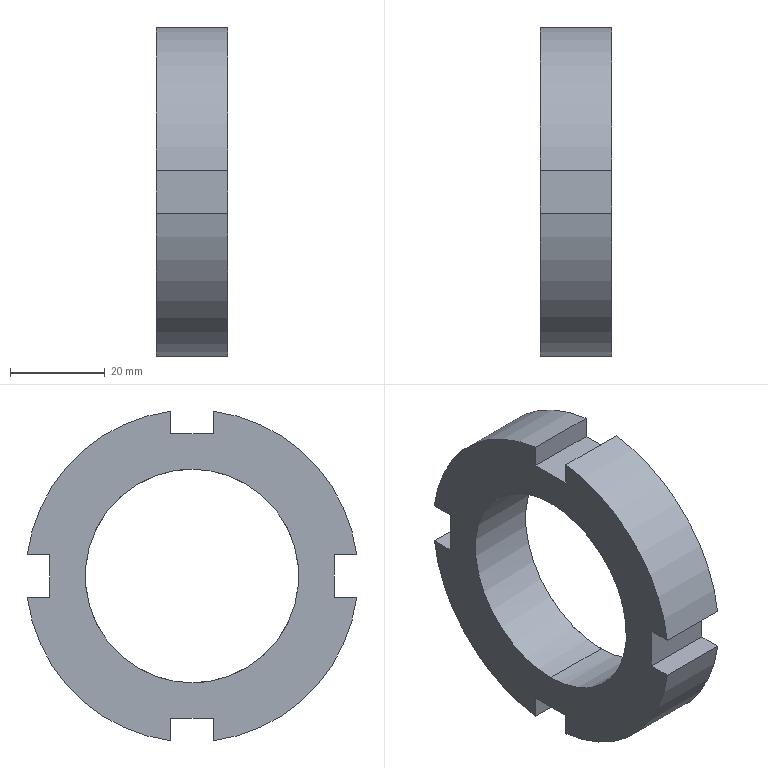Component | SolidWorks | 5Nut-1 | 1 solid | 22 faces | box 15 x 69.42 x 69.42 mm | volume 31223 mm3 | plane 14 | cylinder 6 | cone 2 | commonest cylinder face diameters 70 x4 45 x2
STEP:
#1=COLOUR_RGB('',0.7922,0.8196,0.9333);
#2=FILL_AREA_STYLE_COLOUR('',#1);
#3=FILL_AREA_STYLE('',(#2));
#4=SURFACE_STYLE_FILL_AREA(#3);
#5=SURFACE_SIDE_STYLE('',(#4));
#6=SURFACE_STYLE_USAGE(.BOTH.,#5);
#7=PRESENTATION_STYLE_ASSIGNMENT((#6));
#8=CARTESIAN_POINT('',(-5.674,-3.551,21.043));
#9=VERTEX_POINT('',#8);
#10=CARTESIAN_POINT('',(-5.674,-3.551,19.272));
#11=VERTEX_POINT('',#10);
#12=CARTESIAN_POINT('',(-5.674,-3.551,21.043));
#13=CARTESIAN_POINT('',(-5.674,-3.609,21.043));
#14=CARTESIAN_POINT('',(-5.674,-3.667,21.038));
#15=CARTESIAN_POINT('',(-5.674,-3.781,21.015));
#16=CARTESIAN_POINT('',(-5.674,-3.836,20.998));
#17=CARTESIAN_POINT('',(-5.674,-3.944,20.954));
#18=CARTESIAN_POINT('',(-5.674,-3.995,20.926));
#19=CARTESIAN_POINT('',(-5.674,-4.091,20.862));
#20=CARTESIAN_POINT('',(-5.674,-4.136,20.825));
#21=CARTESIAN_POINT('',(-5.674,-4.218,20.743));
#22=CARTESIAN_POINT('',(-5.674,-4.255,20.698));
#23=CARTESIAN_POINT('',(-5.674,-4.32,20.601));
#24=CARTESIAN_POINT('',(-5.674,-4.347,20.55));
#25=CARTESIAN_POINT('',(-5.674,-4.391,20.443));
#26=CARTESIAN_POINT('',(-5.674,-4.408,20.387));
#27=CARTESIAN_POINT('',(-5.674,-4.431,20.273));
#28=CARTESIAN_POINT('',(-5.674,-4.437,20.216));
#29=CARTESIAN_POINT('',(-5.674,-4.437,20.099));
#30=CARTESIAN_POINT('',(-5.674,-4.431,20.042));
#31=CARTESIAN_POINT('',(-5.674,-4.408,19.928));
#32=CARTESIAN_POINT('',(-5.674,-4.391,19.872));
#33=CARTESIAN_POINT('',(-5.674,-4.347,19.765));
#34=CARTESIAN_POINT('',(-5.674,-4.32,19.714));
#35=CARTESIAN_POINT('',(-5.674,-4.255,19.617));
#36=CARTESIAN_POINT('',(-5.674,-4.218,19.572));
#37=CARTESIAN_POINT('',(-5.674,-4.136,19.49));
#38=CARTESIAN_POINT('',(-5.674,-4.091,19.453));
#39=CARTESIAN_POINT('',(-5.674,-3.995,19.389));
#40=CARTESIAN_POINT('',(-5.674,-3.944,19.361));
#41=CARTESIAN_POINT('',(-5.674,-3.836,19.317));
#42=CARTESIAN_POINT('',(-5.674,-3.781,19.3));
#43=CARTESIAN_POINT('',(-5.674,-3.667,19.277));
#44=CARTESIAN_POINT('',(-5.674,-3.609,19.272));
#45=CARTESIAN_POINT('',(-5.674,-3.551,19.272));
#46=B_SPLINE_CURVE_WITH_KNOTS('',3,(#12,#13,#14,#15,#16,#17,#18,#19,#20,#21,#22,#23,#24,#25,#26,#27,#28,#29,#30,#31,#32,#33,#34,#35,#36,#37,#38,#39,#40,#41,#42,#43,#44,#45),.UNSPECIFIED.,.F.,.F.,(4,2,2,2,2,2,2,2,2,2,2,2,2,2,2,2,4),(0.5,0.5312,0.5625,0.5938,0.625,0.6562,0.6875,0.7188,0.75,0.7812,0.8125,0.8438,0.875,0.9062,0.9375,0.9688,1.),.UNSPECIFIED.);
#47=EDGE_CURVE('',#9,#11,#46,.T.);
#48=ORIENTED_EDGE('',*,*,#47,.F.);
#49=CARTESIAN_POINT('',(-5.084,-3.551,21.043));
#50=VERTEX_POINT('',#49);
#51=CARTESIAN_POINT('',(-5.674,-3.551,21.043));
#52=DIRECTION('',(1.,0.,0.));
#53=VECTOR('',#52,39.37);
#54=LINE('',#51,#53);
#55=EDGE_CURVE('',#9,#50,#54,.T.);
#56=ORIENTED_EDGE('',*,*,#55,.T.);
#57=CARTESIAN_POINT('',(-5.084,-3.551,19.272));
#58=VERTEX_POINT('',#57);
#59=CARTESIAN_POINT('',(-5.084,-3.551,20.157));
#60=DIRECTION('',(-1.,0.,0.));
#61=DIRECTION('',(0.,0.,-1.));
#62=AXIS2_PLACEMENT_3D('',#59,#60,#61);
#63=CIRCLE('',#62,0.8858);
#64=EDGE_CURVE('',#58,#50,#63,.T.);
#65=ORIENTED_EDGE('',*,*,#64,.F.);
#66=CARTESIAN_POINT('',(-5.674,-3.551,19.272));
#67=DIRECTION('',(1.,0.,0.));
#68=VECTOR('',#67,39.37);
#69=LINE('',#66,#68);
#70=EDGE_CURVE('',#11,#58,#69,.T.);
#71=ORIENTED_EDGE('',*,*,#70,.F.);
#72=EDGE_LOOP('',(#48,#56,#65,#71));
#73=FACE_OUTER_BOUND('',#72,.T.);
#74=CARTESIAN_POINT('',(-5.674,-3.551,20.157));
#75=DIRECTION('',(1.,0.,0.));
#76=DIRECTION('',(0.,0.,-1.));
#77=AXIS2_PLACEMENT_3D('',#74,#75,#76);
#78=CYLINDRICAL_SURFACE('',#77,0.8858);
#79=ADVANCED_FACE('',(#73),#78,.F.);
#80=ORIENTED_EDGE('',*,*,#64,.T.);
#81=CARTESIAN_POINT('',(-5.083,-3.551,21.044));
#82=VERTEX_POINT('',#81);
#83=CARTESIAN_POINT('',(-5.083,-3.551,21.044));
#84=DIRECTION('',(0.7071,0.,0.7071));
#85=VECTOR('',#84,39.37);
#86=LINE('',#83,#85);
#87=EDGE_CURVE('',#50,#82,#86,.T.);
#88=ORIENTED_EDGE('',*,*,#87,.T.);
#89=CARTESIAN_POINT('',(-5.083,-3.551,19.271));
#90=VERTEX_POINT('',#89);
#91=CARTESIAN_POINT('',(-5.083,-3.551,20.157));
#92=DIRECTION('',(1.,0.,0.));
#93=DIRECTION('',(0.,0.,-1.));
#94=AXIS2_PLACEMENT_3D('',#91,#92,#93);
#95=CIRCLE('',#94,0.8868);
#96=EDGE_CURVE('',#82,#90,#95,.T.);
#97=ORIENTED_EDGE('',*,*,#96,.T.);
#98=CARTESIAN_POINT('',(-5.083,-3.551,19.271));
#99=DIRECTION('',(0.7071,0.,-0.7071));
#100=VECTOR('',#99,39.37);
#101=LINE('',#98,#100);
#102=EDGE_CURVE('',#58,#90,#101,.T.);
#103=ORIENTED_EDGE('',*,*,#102,.F.);
#104=EDGE_LOOP('',(#80,#88,#97,#103));
#105=FACE_OUTER_BOUND('',#104,.T.);
#106=CARTESIAN_POINT('',(-5.083,-3.551,20.157));
#107=DIRECTION('',(1.,0.,0.));
#108=DIRECTION('',(0.,0.,-1.));
#109=AXIS2_PLACEMENT_3D('',#106,#107,#108);
#110=CONICAL_SURFACE('',#109,0.8868,0.7854);
#111=ADVANCED_FACE('',(#105),#110,.F.);
#112=CARTESIAN_POINT('',(-5.674,-2.184,19.98));
#113=VERTEX_POINT('',#112);
#114=CARTESIAN_POINT('',(-5.083,-2.184,19.98));
#115=VERTEX_POINT('',#114);
#116=CARTESIAN_POINT('',(-5.674,-2.184,19.98));
#117=DIRECTION('',(1.,0.,0.));
#118=VECTOR('',#117,39.37);
#119=LINE('',#116,#118);
#120=EDGE_CURVE('',#113,#115,#119,.T.);
#121=ORIENTED_EDGE('',*,*,#120,.T.);
#122=CARTESIAN_POINT('',(-5.083,-3.374,18.791));
#123=VERTEX_POINT('',#122);
#124=CARTESIAN_POINT('',(-5.083,-3.551,20.157));
#125=DIRECTION('',(1.,0.,0.));
#126=DIRECTION('',(0.,0.,-1.));
#127=AXIS2_PLACEMENT_3D('',#124,#125,#126);
#128=CIRCLE('',#127,1.378);
#129=EDGE_CURVE('',#123,#115,#128,.T.);
#130=ORIENTED_EDGE('',*,*,#129,.F.);
#131=CARTESIAN_POINT('',(-5.674,-3.374,18.791));
#132=VERTEX_POINT('',#131);
#133=CARTESIAN_POINT('',(-5.674,-3.374,18.791));
#134=DIRECTION('',(1.,0.,0.));
#135=VECTOR('',#134,39.37);
#136=LINE('',#133,#135);
#137=EDGE_CURVE('',#132,#123,#136,.T.);
#138=ORIENTED_EDGE('',*,*,#137,.F.);
#139=CARTESIAN_POINT('',(-5.674,-3.551,20.157));
#140=DIRECTION('',(1.,0.,0.));
#141=DIRECTION('',(0.,0.,-1.));
#142=AXIS2_PLACEMENT_3D('',#139,#140,#141);
#143=CIRCLE('',#142,1.378);
#144=EDGE_CURVE('',#132,#113,#143,.T.);
#145=ORIENTED_EDGE('',*,*,#144,.T.);
#146=EDGE_LOOP('',(#121,#130,#138,#145));
#147=FACE_OUTER_BOUND('',#146,.T.);
#148=CARTESIAN_POINT('',(-5.083,-3.551,20.157));
#149=DIRECTION('',(-1.,0.,0.));
#150=DIRECTION('',(0.,0.,1.));
#151=AXIS2_PLACEMENT_3D('',#148,#149,#150);
#152=CYLINDRICAL_SURFACE('',#151,1.378);
#153=ADVANCED_FACE('',(#147),#152,.T.);
#154=CARTESIAN_POINT('',(-5.083,-2.184,20.335));
#155=VERTEX_POINT('',#154);
#156=CARTESIAN_POINT('',(-5.083,-3.374,21.524));
#157=VERTEX_POINT('',#156);
#158=CARTESIAN_POINT('',(-5.083,-3.551,20.157));
#159=DIRECTION('',(1.,0.,0.));
#160=DIRECTION('',(0.,0.,-1.));
#161=AXIS2_PLACEMENT_3D('',#158,#159,#160);
#162=CIRCLE('',#161,1.378);
#163=EDGE_CURVE('',#155,#157,#162,.T.);
#164=ORIENTED_EDGE('',*,*,#163,.F.);
#165=CARTESIAN_POINT('',(-5.674,-2.184,20.335));
#166=VERTEX_POINT('',#165);
#167=CARTESIAN_POINT('',(-5.674,-2.184,20.335));
#168=DIRECTION('',(1.,0.,0.));
#169=VECTOR('',#168,39.37);
#170=LINE('',#167,#169);
#171=EDGE_CURVE('',#166,#155,#170,.T.);
#172=ORIENTED_EDGE('',*,*,#171,.F.);
#173=CARTESIAN_POINT('',(-5.674,-3.374,21.524));
#174=VERTEX_POINT('',#173);
#175=CARTESIAN_POINT('',(-5.674,-3.551,20.157));
#176=DIRECTION('',(1.,0.,0.));
#177=DIRECTION('',(0.,0.,-1.));
#178=AXIS2_PLACEMENT_3D('',#175,#176,#177);
#179=CIRCLE('',#178,1.378);
#180=EDGE_CURVE('',#166,#174,#179,.T.);
#181=ORIENTED_EDGE('',*,*,#180,.T.);
#182=CARTESIAN_POINT('',(-5.674,-3.374,21.524));
#183=DIRECTION('',(1.,0.,0.));
#184=VECTOR('',#183,39.37);
#185=LINE('',#182,#184);
#186=EDGE_CURVE('',#174,#157,#185,.T.);
#187=ORIENTED_EDGE('',*,*,#186,.T.);
#188=EDGE_LOOP('',(#164,#172,#181,#187));
#189=FACE_OUTER_BOUND('',#188,.T.);
#190=CARTESIAN_POINT('',(-5.083,-3.551,20.157));
#191=DIRECTION('',(-1.,0.,0.));
#192=DIRECTION('',(0.,0.,1.));
#193=AXIS2_PLACEMENT_3D('',#190,#191,#192);
#194=CYLINDRICAL_SURFACE('',#193,1.378);
#195=ADVANCED_FACE('',(#189),#194,.T.);
#196=CARTESIAN_POINT('',(-5.083,-3.728,21.524));
#197=VERTEX_POINT('',#196);
#198=CARTESIAN_POINT('',(-5.083,-4.917,20.335));
#199=VERTEX_POINT('',#198);
#200=CARTESIAN_POINT('',(-5.083,-3.551,20.157));
#201=DIRECTION('',(1.,0.,0.));
#202=DIRECTION('',(0.,0.,-1.));
#203=AXIS2_PLACEMENT_3D('',#200,#201,#202);
#204=CIRCLE('',#203,1.378);
#205=EDGE_CURVE('',#197,#199,#204,.T.);
#206=ORIENTED_EDGE('',*,*,#205,.F.);
#207=CARTESIAN_POINT('',(-5.674,-3.728,21.524));
#208=VERTEX_POINT('',#207);
#209=CARTESIAN_POINT('',(-5.674,-3.728,21.524));
#210=DIRECTION('',(1.,0.,0.));
#211=VECTOR('',#210,39.37);
#212=LINE('',#209,#211);
#213=EDGE_CURVE('',#208,#197,#212,.T.);
#214=ORIENTED_EDGE('',*,*,#213,.F.);
#215=CARTESIAN_POINT('',(-5.674,-4.917,20.335));
#216=VERTEX_POINT('',#215);
#217=CARTESIAN_POINT('',(-5.674,-3.551,20.157));
#218=DIRECTION('',(1.,0.,0.));
#219=DIRECTION('',(0.,0.,-1.));
#220=AXIS2_PLACEMENT_3D('',#217,#218,#219);
#221=CIRCLE('',#220,1.378);
#222=EDGE_CURVE('',#208,#216,#221,.T.);
#223=ORIENTED_EDGE('',*,*,#222,.T.);
#224=CARTESIAN_POINT('',(-5.674,-4.917,20.335));
#225=DIRECTION('',(1.,0.,0.));
#226=VECTOR('',#225,39.37);
#227=LINE('',#224,#226);
#228=EDGE_CURVE('',#216,#199,#227,.T.);
#229=ORIENTED_EDGE('',*,*,#228,.T.);
#230=EDGE_LOOP('',(#206,#214,#223,#229));
#231=FACE_OUTER_BOUND('',#230,.T.);
#232=CARTESIAN_POINT('',(-5.083,-3.551,20.157));
#233=DIRECTION('',(-1.,0.,0.));
#234=DIRECTION('',(0.,0.,1.));
#235=AXIS2_PLACEMENT_3D('',#232,#233,#234);
#236=CYLINDRICAL_SURFACE('',#235,1.378);
#237=ADVANCED_FACE('',(#231),#236,.T.);
#238=CARTESIAN_POINT('',(-5.083,-4.917,19.98));
#239=VERTEX_POINT('',#238);
#240=CARTESIAN_POINT('',(-5.083,-3.728,18.791));
#241=VERTEX_POINT('',#240);
#242=CARTESIAN_POINT('',(-5.083,-3.551,20.157));
#243=DIRECTION('',(1.,0.,0.));
#244=DIRECTION('',(0.,0.,-1.));
#245=AXIS2_PLACEMENT_3D('',#242,#243,#244);
#246=CIRCLE('',#245,1.378);
#247=EDGE_CURVE('',#239,#241,#246,.T.);
#248=ORIENTED_EDGE('',*,*,#247,.F.);
#249=CARTESIAN_POINT('',(-5.674,-4.917,19.98));
#250=VERTEX_POINT('',#249);
#251=CARTESIAN_POINT('',(-5.674,-4.917,19.98));
#252=DIRECTION('',(1.,0.,0.));
#253=VECTOR('',#252,39.37);
#254=LINE('',#251,#253);
#255=EDGE_CURVE('',#250,#239,#254,.T.);
#256=ORIENTED_EDGE('',*,*,#255,.F.);
#257=CARTESIAN_POINT('',(-5.674,-3.728,18.791));
#258=VERTEX_POINT('',#257);
#259=CARTESIAN_POINT('',(-5.674,-3.551,20.157));
#260=DIRECTION('',(1.,0.,0.));
#261=DIRECTION('',(0.,0.,-1.));
#262=AXIS2_PLACEMENT_3D('',#259,#260,#261);
#263=CIRCLE('',#262,1.378);
#264=EDGE_CURVE('',#250,#258,#263,.T.);
#265=ORIENTED_EDGE('',*,*,#264,.T.);
#266=CARTESIAN_POINT('',(-5.674,-3.728,18.791));
#267=DIRECTION('',(1.,0.,0.));
#268=VECTOR('',#267,39.37);
#269=LINE('',#266,#268);
#270=EDGE_CURVE('',#258,#241,#269,.T.);
#271=ORIENTED_EDGE('',*,*,#270,.T.);
#272=EDGE_LOOP('',(#248,#256,#265,#271));
#273=FACE_OUTER_BOUND('',#272,.T.);
#274=CARTESIAN_POINT('',(-5.083,-3.551,20.157));
#275=DIRECTION('',(-1.,0.,0.));
#276=DIRECTION('',(0.,0.,1.));
#277=AXIS2_PLACEMENT_3D('',#274,#275,#276);
#278=CYLINDRICAL_SURFACE('',#277,1.378);
#279=ADVANCED_FACE('',(#273),#278,.T.);
#280=CARTESIAN_POINT('',(-5.083,-3.551,20.157));
#281=DIRECTION('',(1.,0.,0.));
#282=DIRECTION('',(0.,0.,-1.));
#283=AXIS2_PLACEMENT_3D('',#280,#281,#282);
#284=CIRCLE('',#283,0.8868);
#285=EDGE_CURVE('',#90,#82,#284,.T.);
#286=ORIENTED_EDGE('',*,*,#285,.F.);
#287=ORIENTED_EDGE('',*,*,#96,.F.);
#288=EDGE_LOOP('',(#286,#287));
#289=FACE_BOUND('',#288,.T.);
#290=CARTESIAN_POINT('',(-5.083,-2.37,20.335));
#291=VERTEX_POINT('',#290);
#292=CARTESIAN_POINT('',(-5.083,-3.551,20.335));
#293=DIRECTION('',(0.,-1.,-0.));
#294=VECTOR('',#293,39.37);
#295=LINE('',#292,#294);
#296=EDGE_CURVE('',#155,#291,#295,.T.);
#297=ORIENTED_EDGE('',*,*,#296,.F.);
#298=ORIENTED_EDGE('',*,*,#163,.T.);
#299=CARTESIAN_POINT('',(-5.083,-3.374,21.339));
#300=VERTEX_POINT('',#299);
#301=CARTESIAN_POINT('',(-5.083,-3.374,20.157));
#302=DIRECTION('',(0.,0.,-1.));
#303=VECTOR('',#302,39.37);
#304=LINE('',#301,#303);
#305=EDGE_CURVE('',#157,#300,#304,.T.);
#306=ORIENTED_EDGE('',*,*,#305,.T.);
#307=CARTESIAN_POINT('',(-5.083,-3.728,21.339));
#308=VERTEX_POINT('',#307);
#309=CARTESIAN_POINT('',(-5.083,-3.551,21.339));
#310=DIRECTION('',(0.,1.,0.));
#311=VECTOR('',#310,39.37);
#312=LINE('',#309,#311);
#313=EDGE_CURVE('',#308,#300,#312,.T.);
#314=ORIENTED_EDGE('',*,*,#313,.F.);
#315=CARTESIAN_POINT('',(-5.083,-3.728,20.157));
#316=DIRECTION('',(0.,-0.,-1.));
#317=VECTOR('',#316,39.37);
#318=LINE('',#315,#317);
#319=EDGE_CURVE('',#197,#308,#318,.T.);
#320=ORIENTED_EDGE('',*,*,#319,.F.);
#321=ORIENTED_EDGE('',*,*,#205,.T.);
#322=CARTESIAN_POINT('',(-5.083,-4.732,20.335));
#323=VERTEX_POINT('',#322);
#324=CARTESIAN_POINT('',(-5.083,-3.551,20.335));
#325=DIRECTION('',(0.,1.,0.));
#326=VECTOR('',#325,39.37);
#327=LINE('',#324,#326);
#328=EDGE_CURVE('',#199,#323,#327,.T.);
#329=ORIENTED_EDGE('',*,*,#328,.T.);
#330=CARTESIAN_POINT('',(-5.083,-4.732,19.98));
#331=VERTEX_POINT('',#330);
#332=CARTESIAN_POINT('',(-5.083,-4.732,20.157));
#333=DIRECTION('',(0.,-0.,1.));
#334=VECTOR('',#333,39.37);
#335=LINE('',#332,#334);
#336=EDGE_CURVE('',#331,#323,#335,.T.);
#337=ORIENTED_EDGE('',*,*,#336,.F.);
#338=CARTESIAN_POINT('',(-5.083,-3.551,19.98));
#339=DIRECTION('',(0.,1.,0.));
#340=VECTOR('',#339,39.37);
#341=LINE('',#338,#340);
#342=EDGE_CURVE('',#239,#331,#341,.T.);
#343=ORIENTED_EDGE('',*,*,#342,.F.);
#344=ORIENTED_EDGE('',*,*,#247,.T.);
#345=CARTESIAN_POINT('',(-5.083,-3.728,18.976));
#346=VERTEX_POINT('',#345);
#347=CARTESIAN_POINT('',(-5.083,-3.728,20.157));
#348=DIRECTION('',(0.,-0.,1.));
#349=VECTOR('',#348,39.37);
#350=LINE('',#347,#349);
#351=EDGE_CURVE('',#241,#346,#350,.T.);
#352=ORIENTED_EDGE('',*,*,#351,.T.);
#353=CARTESIAN_POINT('',(-5.083,-3.374,18.976));
#354=VERTEX_POINT('',#353);
#355=CARTESIAN_POINT('',(-5.083,-3.551,18.976));
#356=DIRECTION('',(0.,-1.,0.));
#357=VECTOR('',#356,39.37);
#358=LINE('',#355,#357);
#359=EDGE_CURVE('',#354,#346,#358,.T.);
#360=ORIENTED_EDGE('',*,*,#359,.F.);
#361=CARTESIAN_POINT('',(-5.083,-3.374,20.157));
#362=DIRECTION('',(0.,0.,1.));
#363=VECTOR('',#362,39.37);
#364=LINE('',#361,#363);
#365=EDGE_CURVE('',#123,#354,#364,.T.);
#366=ORIENTED_EDGE('',*,*,#365,.F.);
#367=ORIENTED_EDGE('',*,*,#129,.T.);
#368=CARTESIAN_POINT('',(-5.083,-2.37,19.98));
#369=VERTEX_POINT('',#368);
#370=CARTESIAN_POINT('',(-5.083,-3.551,19.98));
#371=DIRECTION('',(0.,-1.,-0.));
#372=VECTOR('',#371,39.37);
#373=LINE('',#370,#372);
#374=EDGE_CURVE('',#115,#369,#373,.T.);
#375=ORIENTED_EDGE('',*,*,#374,.T.);
#376=CARTESIAN_POINT('',(-5.083,-2.37,20.157));
#377=DIRECTION('',(0.,0.,-1.));
#378=VECTOR('',#377,39.37);
#379=LINE('',#376,#378);
#380=EDGE_CURVE('',#291,#369,#379,.T.);
#381=ORIENTED_EDGE('',*,*,#380,.F.);
#382=EDGE_LOOP('',(#297,#298,#306,#314,#320,#321,#329,#337,#343,#344,#352,#360,#366,#367,#375,#381));
#383=FACE_OUTER_BOUND('',#382,.T.);
#384=CARTESIAN_POINT('',(-5.083,-3.551,20.157));
#385=DIRECTION('',(1.,0.,0.));
#386=DIRECTION('',(0.,0.,-1.));
#387=AXIS2_PLACEMENT_3D('',#384,#385,#386);
#388=PLANE('',#387);
#389=ADVANCED_FACE('',(#289,#383),#388,.T.);
#390=CARTESIAN_POINT('',(-5.674,-3.551,19.272));
#391=CARTESIAN_POINT('',(-5.674,-3.493,19.272));
#392=CARTESIAN_POINT('',(-5.674,-3.435,19.277));
#393=CARTESIAN_POINT('',(-5.674,-3.321,19.3));
#394=CARTESIAN_POINT('',(-5.674,-3.266,19.317));
#395=CARTESIAN_POINT('',(-5.674,-3.158,19.361));
#396=CARTESIAN_POINT('',(-5.674,-3.107,19.389));
#397=CARTESIAN_POINT('',(-5.674,-3.01,19.453));
#398=CARTESIAN_POINT('',(-5.674,-2.966,19.49));
#399=CARTESIAN_POINT('',(-5.674,-2.883,19.572));
#400=CARTESIAN_POINT('',(-5.674,-2.847,19.617));
#401=CARTESIAN_POINT('',(-5.674,-2.782,19.714));
#402=CARTESIAN_POINT('',(-5.674,-2.755,19.765));
#403=CARTESIAN_POINT('',(-5.674,-2.71,19.872));
#404=CARTESIAN_POINT('',(-5.674,-2.693,19.928));
#405=CARTESIAN_POINT('',(-5.674,-2.671,20.042));
#406=CARTESIAN_POINT('',(-5.674,-2.665,20.099));
#407=CARTESIAN_POINT('',(-5.674,-2.665,20.216));
#408=CARTESIAN_POINT('',(-5.674,-2.671,20.273));
#409=CARTESIAN_POINT('',(-5.674,-2.693,20.387));
#410=CARTESIAN_POINT('',(-5.674,-2.71,20.443));
#411=CARTESIAN_POINT('',(-5.674,-2.755,20.55));
#412=CARTESIAN_POINT('',(-5.674,-2.782,20.601));
#413=CARTESIAN_POINT('',(-5.674,-2.847,20.698));
#414=CARTESIAN_POINT('',(-5.674,-2.883,20.743));
#415=CARTESIAN_POINT('',(-5.674,-2.966,20.825));
#416=CARTESIAN_POINT('',(-5.674,-3.01,20.862));
#417=CARTESIAN_POINT('',(-5.674,-3.107,20.926));
#418=CARTESIAN_POINT('',(-5.674,-3.158,20.954));
#419=CARTESIAN_POINT('',(-5.674,-3.266,20.998));
#420=CARTESIAN_POINT('',(-5.674,-3.321,21.015));
#421=CARTESIAN_POINT('',(-5.674,-3.435,21.038));
#422=CARTESIAN_POINT('',(-5.674,-3.493,21.043));
#423=CARTESIAN_POINT('',(-5.674,-3.551,21.043));
#424=B_SPLINE_CURVE_WITH_KNOTS('',3,(#390,#391,#392,#393,#394,#395,#396,#397,#398,#399,#400,#401,#402,#403,#404,#405,#406,#407,#408,#409,#410,#411,#412,#413,#414,#415,#416,#417,#418,#419,#420,#421,#422,#423),.UNSPECIFIED.,.F.,.F.,(4,2,2,2,2,2,2,2,2,2,2,2,2,2,2,2,4),(0.,0.03125,0.0625,0.09375,0.125,0.1562,0.1875,0.2187,0.25,0.2812,0.3125,0.3437,0.375,0.4062,0.4375,0.4687,0.5),.UNSPECIFIED.);
#425=EDGE_CURVE('',#11,#9,#424,.T.);
#426=ORIENTED_EDGE('',*,*,#425,.T.);
#427=ORIENTED_EDGE('',*,*,#47,.T.);
#428=EDGE_LOOP('',(#426,#427));
#429=FACE_BOUND('',#428,.T.);
#430=ORIENTED_EDGE('',*,*,#180,.F.);
#431=CARTESIAN_POINT('',(-5.674,-2.37,20.335));
#432=VERTEX_POINT('',#431);
#433=CARTESIAN_POINT('',(-5.674,-3.551,20.335));
#434=DIRECTION('',(0.,-1.,-0.));
#435=VECTOR('',#434,39.37);
#436=LINE('',#433,#435);
#437=EDGE_CURVE('',#166,#432,#436,.T.);
#438=ORIENTED_EDGE('',*,*,#437,.T.);
#439=CARTESIAN_POINT('',(-5.674,-2.37,19.98));
#440=VERTEX_POINT('',#439);
#441=CARTESIAN_POINT('',(-5.674,-2.37,20.157));
#442=DIRECTION('',(0.,0.,-1.));
#443=VECTOR('',#442,39.37);
#444=LINE('',#441,#443);
#445=EDGE_CURVE('',#432,#440,#444,.T.);
#446=ORIENTED_EDGE('',*,*,#445,.T.);
#447=CARTESIAN_POINT('',(-5.674,-3.551,19.98));
#448=DIRECTION('',(0.,-1.,-0.));
#449=VECTOR('',#448,39.37);
#450=LINE('',#447,#449);
#451=EDGE_CURVE('',#113,#440,#450,.T.);
#452=ORIENTED_EDGE('',*,*,#451,.F.);
#453=ORIENTED_EDGE('',*,*,#144,.F.);
#454=CARTESIAN_POINT('',(-5.674,-3.374,18.976));
#455=VERTEX_POINT('',#454);
#456=CARTESIAN_POINT('',(-5.674,-3.374,20.157));
#457=DIRECTION('',(0.,0.,1.));
#458=VECTOR('',#457,39.37);
#459=LINE('',#456,#458);
#460=EDGE_CURVE('',#132,#455,#459,.T.);
#461=ORIENTED_EDGE('',*,*,#460,.T.);
#462=CARTESIAN_POINT('',(-5.674,-3.728,18.976));
#463=VERTEX_POINT('',#462);
#464=CARTESIAN_POINT('',(-5.674,-3.551,18.976));
#465=DIRECTION('',(0.,-1.,0.));
#466=VECTOR('',#465,39.37);
#467=LINE('',#464,#466);
#468=EDGE_CURVE('',#455,#463,#467,.T.);
#469=ORIENTED_EDGE('',*,*,#468,.T.);
#470=CARTESIAN_POINT('',(-5.674,-3.728,20.157));
#471=DIRECTION('',(0.,-0.,1.));
#472=VECTOR('',#471,39.37);
#473=LINE('',#470,#472);
#474=EDGE_CURVE('',#258,#463,#473,.T.);
#475=ORIENTED_EDGE('',*,*,#474,.F.);
#476=ORIENTED_EDGE('',*,*,#264,.F.);
#477=CARTESIAN_POINT('',(-5.674,-4.732,19.98));
#478=VERTEX_POINT('',#477);
#479=CARTESIAN_POINT('',(-5.674,-3.551,19.98));
#480=DIRECTION('',(0.,1.,0.));
#481=VECTOR('',#480,39.37);
#482=LINE('',#479,#481);
#483=EDGE_CURVE('',#250,#478,#482,.T.);
#484=ORIENTED_EDGE('',*,*,#483,.T.);
#485=CARTESIAN_POINT('',(-5.674,-4.732,20.335));
#486=VERTEX_POINT('',#485);
#487=CARTESIAN_POINT('',(-5.674,-4.732,20.157));
#488=DIRECTION('',(0.,-0.,1.));
#489=VECTOR('',#488,39.37);
#490=LINE('',#487,#489);
#491=EDGE_CURVE('',#478,#486,#490,.T.);
#492=ORIENTED_EDGE('',*,*,#491,.T.);
#493=CARTESIAN_POINT('',(-5.674,-3.551,20.335));
#494=DIRECTION('',(0.,1.,0.));
#495=VECTOR('',#494,39.37);
#496=LINE('',#493,#495);
#497=EDGE_CURVE('',#216,#486,#496,.T.);
#498=ORIENTED_EDGE('',*,*,#497,.F.);
#499=ORIENTED_EDGE('',*,*,#222,.F.);
#500=CARTESIAN_POINT('',(-5.674,-3.728,21.339));
#501=VERTEX_POINT('',#500);
#502=CARTESIAN_POINT('',(-5.674,-3.728,20.157));
#503=DIRECTION('',(0.,-0.,-1.));
#504=VECTOR('',#503,39.37);
#505=LINE('',#502,#504);
#506=EDGE_CURVE('',#208,#501,#505,.T.);
#507=ORIENTED_EDGE('',*,*,#506,.T.);
#508=CARTESIAN_POINT('',(-5.674,-3.374,21.339));
#509=VERTEX_POINT('',#508);
#510=CARTESIAN_POINT('',(-5.674,-3.551,21.339));
#511=DIRECTION('',(0.,1.,0.));
#512=VECTOR('',#511,39.37);
#513=LINE('',#510,#512);
#514=EDGE_CURVE('',#501,#509,#513,.T.);
#515=ORIENTED_EDGE('',*,*,#514,.T.);
#516=CARTESIAN_POINT('',(-5.674,-3.374,20.157));
#517=DIRECTION('',(0.,0.,-1.));
#518=VECTOR('',#517,39.37);
#519=LINE('',#516,#518);
#520=EDGE_CURVE('',#174,#509,#519,.T.);
#521=ORIENTED_EDGE('',*,*,#520,.F.);
#522=EDGE_LOOP('',(#430,#438,#446,#452,#453,#461,#469,#475,#476,#484,#492,#498,#499,#507,#515,#521));
#523=FACE_OUTER_BOUND('',#522,.T.);
#524=CARTESIAN_POINT('',(-5.674,-3.551,20.157));
#525=DIRECTION('',(1.,0.,0.));
#526=DIRECTION('',(0.,0.,-1.));
#527=AXIS2_PLACEMENT_3D('',#524,#525,#526);
#528=PLANE('',#527);
#529=ADVANCED_FACE('',(#429,#523),#528,.F.);
#530=ORIENTED_EDGE('',*,*,#359,.T.);
#531=CARTESIAN_POINT('',(-5.674,-3.728,18.976));
#532=DIRECTION('',(1.,0.,0.));
#533=VECTOR('',#532,39.37);
#534=LINE('',#531,#533);
#535=EDGE_CURVE('',#463,#346,#534,.T.);
#536=ORIENTED_EDGE('',*,*,#535,.F.);
#537=ORIENTED_EDGE('',*,*,#468,.F.);
#538=CARTESIAN_POINT('',(-5.674,-3.374,18.976));
#539=DIRECTION('',(1.,0.,0.));
#540=VECTOR('',#539,39.37);
#541=LINE('',#538,#540);
#542=EDGE_CURVE('',#455,#354,#541,.T.);
#543=ORIENTED_EDGE('',*,*,#542,.T.);
#544=EDGE_LOOP('',(#530,#536,#537,#543));
#545=FACE_OUTER_BOUND('',#544,.T.);
#546=CARTESIAN_POINT('',(-5.674,-3.551,18.976));
#547=DIRECTION('',(0.,0.,1.));
#548=DIRECTION('',(1.,0.,0.));
#549=AXIS2_PLACEMENT_3D('',#546,#547,#548);
#550=PLANE('',#549);
#551=ADVANCED_FACE('',(#545),#550,.F.);
#552=ORIENTED_EDGE('',*,*,#365,.T.);
#553=ORIENTED_EDGE('',*,*,#542,.F.);
#554=ORIENTED_EDGE('',*,*,#460,.F.);
#555=ORIENTED_EDGE('',*,*,#137,.T.);
#556=EDGE_LOOP('',(#552,#553,#554,#555));
#557=FACE_OUTER_BOUND('',#556,.T.);
#558=CARTESIAN_POINT('',(-5.674,-3.374,20.157));
#559=DIRECTION('',(0.,1.,-0.));
#560=DIRECTION('',(0.,0.,1.));
#561=AXIS2_PLACEMENT_3D('',#558,#559,#560);
#562=PLANE('',#561);
#563=ADVANCED_FACE('',(#557),#562,.F.);
#564=ORIENTED_EDGE('',*,*,#351,.F.);
#565=ORIENTED_EDGE('',*,*,#270,.F.);
#566=ORIENTED_EDGE('',*,*,#474,.T.);
#567=ORIENTED_EDGE('',*,*,#535,.T.);
#568=EDGE_LOOP('',(#564,#565,#566,#567));
#569=FACE_OUTER_BOUND('',#568,.T.);
#570=CARTESIAN_POINT('',(-5.674,-3.728,20.157));
#571=DIRECTION('',(0.,1.,0.));
#572=DIRECTION('',(0.,-0.,1.));
#573=AXIS2_PLACEMENT_3D('',#570,#571,#572);
#574=PLANE('',#573);
#575=ADVANCED_FACE('',(#569),#574,.T.);
#576=ORIENTED_EDGE('',*,*,#336,.T.);
#577=CARTESIAN_POINT('',(-5.674,-4.732,20.335));
#578=DIRECTION('',(1.,0.,0.));
#579=VECTOR('',#578,39.37);
#580=LINE('',#577,#579);
#581=EDGE_CURVE('',#486,#323,#580,.T.);
#582=ORIENTED_EDGE('',*,*,#581,.F.);
#583=ORIENTED_EDGE('',*,*,#491,.F.);
#584=CARTESIAN_POINT('',(-5.674,-4.732,19.98));
#585=DIRECTION('',(1.,0.,0.));
#586=VECTOR('',#585,39.37);
#587=LINE('',#584,#586);
#588=EDGE_CURVE('',#478,#331,#587,.T.);
#589=ORIENTED_EDGE('',*,*,#588,.T.);
#590=EDGE_LOOP('',(#576,#582,#583,#589));
#591=FACE_OUTER_BOUND('',#590,.T.);
#592=CARTESIAN_POINT('',(-5.674,-4.732,20.157));
#593=DIRECTION('',(0.,1.,0.));
#594=DIRECTION('',(0.,-0.,1.));
#595=AXIS2_PLACEMENT_3D('',#592,#593,#594);
#596=PLANE('',#595);
#597=ADVANCED_FACE('',(#591),#596,.F.);
#598=ORIENTED_EDGE('',*,*,#342,.T.);
#599=ORIENTED_EDGE('',*,*,#588,.F.);
#600=ORIENTED_EDGE('',*,*,#483,.F.);
#601=ORIENTED_EDGE('',*,*,#255,.T.);
#602=EDGE_LOOP('',(#598,#599,#600,#601));
#603=FACE_OUTER_BOUND('',#602,.T.);
#604=CARTESIAN_POINT('',(-5.674,-3.551,19.98));
#605=DIRECTION('',(0.,0.,-1.));
#606=DIRECTION('',(0.,1.,0.));
#607=AXIS2_PLACEMENT_3D('',#604,#605,#606);
#608=PLANE('',#607);
#609=ADVANCED_FACE('',(#603),#608,.F.);
#610=ORIENTED_EDGE('',*,*,#328,.F.);
#611=ORIENTED_EDGE('',*,*,#228,.F.);
#612=ORIENTED_EDGE('',*,*,#497,.T.);
#613=ORIENTED_EDGE('',*,*,#581,.T.);
#614=EDGE_LOOP('',(#610,#611,#612,#613));
#615=FACE_OUTER_BOUND('',#614,.T.);
#616=CARTESIAN_POINT('',(-5.674,-3.551,20.335));
#617=DIRECTION('',(0.,0.,-1.));
#618=DIRECTION('',(0.,1.,0.));
#619=AXIS2_PLACEMENT_3D('',#616,#617,#618);
#620=PLANE('',#619);
#621=ADVANCED_FACE('',(#615),#620,.T.);
#622=ORIENTED_EDGE('',*,*,#313,.T.);
#623=CARTESIAN_POINT('',(-5.674,-3.374,21.339));
#624=DIRECTION('',(1.,0.,0.));
#625=VECTOR('',#624,39.37);
#626=LINE('',#623,#625);
#627=EDGE_CURVE('',#509,#300,#626,.T.);
#628=ORIENTED_EDGE('',*,*,#627,.F.);
#629=ORIENTED_EDGE('',*,*,#514,.F.);
#630=CARTESIAN_POINT('',(-5.674,-3.728,21.339));
#631=DIRECTION('',(1.,0.,0.));
#632=VECTOR('',#631,39.37);
#633=LINE('',#630,#632);
#634=EDGE_CURVE('',#501,#308,#633,.T.);
#635=ORIENTED_EDGE('',*,*,#634,.T.);
#636=EDGE_LOOP('',(#622,#628,#629,#635));
#637=FACE_OUTER_BOUND('',#636,.T.);
#638=CARTESIAN_POINT('',(-5.674,-3.551,21.339));
#639=DIRECTION('',(0.,0.,-1.));
#640=DIRECTION('',(-1.,0.,0.));
#641=AXIS2_PLACEMENT_3D('',#638,#639,#640);
#642=PLANE('',#641);
#643=ADVANCED_FACE('',(#637),#642,.F.);
#644=ORIENTED_EDGE('',*,*,#319,.T.);
#645=ORIENTED_EDGE('',*,*,#634,.F.);
#646=ORIENTED_EDGE('',*,*,#506,.F.);
#647=ORIENTED_EDGE('',*,*,#213,.T.);
#648=EDGE_LOOP('',(#644,#645,#646,#647));
#649=FACE_OUTER_BOUND('',#648,.T.);
#650=CARTESIAN_POINT('',(-5.674,-3.728,20.157));
#651=DIRECTION('',(0.,-1.,0.));
#652=DIRECTION('',(0.,-0.,-1.));
#653=AXIS2_PLACEMENT_3D('',#650,#651,#652);
#654=PLANE('',#653);
#655=ADVANCED_FACE('',(#649),#654,.F.);
#656=ORIENTED_EDGE('',*,*,#305,.F.);
#657=ORIENTED_EDGE('',*,*,#186,.F.);
#658=ORIENTED_EDGE('',*,*,#520,.T.);
#659=ORIENTED_EDGE('',*,*,#627,.T.);
#660=EDGE_LOOP('',(#656,#657,#658,#659));
#661=FACE_OUTER_BOUND('',#660,.T.);
#662=CARTESIAN_POINT('',(-5.674,-3.374,20.157));
#663=DIRECTION('',(0.,-1.,-0.));
#664=DIRECTION('',(0.,0.,-1.));
#665=AXIS2_PLACEMENT_3D('',#662,#663,#664);
#666=PLANE('',#665);
#667=ADVANCED_FACE('',(#661),#666,.T.);
#668=ORIENTED_EDGE('',*,*,#380,.T.);
#669=CARTESIAN_POINT('',(-5.674,-2.37,19.98));
#670=DIRECTION('',(1.,0.,0.));
#671=VECTOR('',#670,39.37);
#672=LINE('',#669,#671);
#673=EDGE_CURVE('',#440,#369,#672,.T.);
#674=ORIENTED_EDGE('',*,*,#673,.F.);
#675=ORIENTED_EDGE('',*,*,#445,.F.);
#676=CARTESIAN_POINT('',(-5.674,-2.37,20.335));
#677=DIRECTION('',(1.,0.,0.));
#678=VECTOR('',#677,39.37);
#679=LINE('',#676,#678);
#680=EDGE_CURVE('',#432,#291,#679,.T.);
#681=ORIENTED_EDGE('',*,*,#680,.T.);
#682=EDGE_LOOP('',(#668,#674,#675,#681));
#683=FACE_OUTER_BOUND('',#682,.T.);
#684=CARTESIAN_POINT('',(-5.674,-2.37,20.157));
#685=DIRECTION('',(0.,-1.,-0.));
#686=DIRECTION('',(0.,0.,-1.));
#687=AXIS2_PLACEMENT_3D('',#684,#685,#686);
#688=PLANE('',#687);
#689=ADVANCED_FACE('',(#683),#688,.F.);
#690=ORIENTED_EDGE('',*,*,#296,.T.);
#691=ORIENTED_EDGE('',*,*,#680,.F.);
#692=ORIENTED_EDGE('',*,*,#437,.F.);
#693=ORIENTED_EDGE('',*,*,#171,.T.);
#694=EDGE_LOOP('',(#690,#691,#692,#693));
#695=FACE_OUTER_BOUND('',#694,.T.);
#696=CARTESIAN_POINT('',(-5.674,-3.551,20.335));
#697=DIRECTION('',(0.,-0.,1.));
#698=DIRECTION('',(0.,-1.,-0.));
#699=AXIS2_PLACEMENT_3D('',#696,#697,#698);
#700=PLANE('',#699);
#701=ADVANCED_FACE('',(#695),#700,.F.);
#702=ORIENTED_EDGE('',*,*,#374,.F.);
#703=ORIENTED_EDGE('',*,*,#120,.F.);
#704=ORIENTED_EDGE('',*,*,#451,.T.);
#705=ORIENTED_EDGE('',*,*,#673,.T.);
#706=EDGE_LOOP('',(#702,#703,#704,#705));
#707=FACE_OUTER_BOUND('',#706,.T.);
#708=CARTESIAN_POINT('',(-5.674,-3.551,19.98));
#709=DIRECTION('',(0.,-0.,1.));
#710=DIRECTION('',(0.,-1.,-0.));
#711=AXIS2_PLACEMENT_3D('',#708,#709,#710);
#712=PLANE('',#711);
#713=ADVANCED_FACE('',(#707),#712,.T.);
#714=ORIENTED_EDGE('',*,*,#87,.F.);
#715=CARTESIAN_POINT('',(-5.084,-3.551,20.157));
#716=DIRECTION('',(-1.,0.,0.));
#717=DIRECTION('',(0.,0.,-1.));
#718=AXIS2_PLACEMENT_3D('',#715,#716,#717);
#719=CIRCLE('',#718,0.8858);
#720=EDGE_CURVE('',#50,#58,#719,.T.);
#721=ORIENTED_EDGE('',*,*,#720,.T.);
#722=ORIENTED_EDGE('',*,*,#102,.T.);
#723=ORIENTED_EDGE('',*,*,#285,.T.);
#724=EDGE_LOOP('',(#714,#721,#722,#723));
#725=FACE_OUTER_BOUND('',#724,.T.);
#726=CARTESIAN_POINT('',(-5.083,-3.551,20.157));
#727=DIRECTION('',(1.,0.,0.));
#728=DIRECTION('',(0.,0.,-1.));
#729=AXIS2_PLACEMENT_3D('',#726,#727,#728);
#730=CONICAL_SURFACE('',#729,0.8868,0.7854);
#731=ADVANCED_FACE('',(#725),#730,.F.);
#732=ORIENTED_EDGE('',*,*,#55,.F.);
#733=ORIENTED_EDGE('',*,*,#425,.F.);
#734=ORIENTED_EDGE('',*,*,#70,.T.);
#735=ORIENTED_EDGE('',*,*,#720,.F.);
#736=EDGE_LOOP('',(#732,#733,#734,#735));
#737=FACE_OUTER_BOUND('',#736,.T.);
#738=CARTESIAN_POINT('',(-5.674,-3.551,20.157));
#739=DIRECTION('',(1.,0.,0.));
#740=DIRECTION('',(0.,0.,-1.));
#741=AXIS2_PLACEMENT_3D('',#738,#739,#740);
#742=CYLINDRICAL_SURFACE('',#741,0.8858);
#743=ADVANCED_FACE('',(#737),#742,.F.);
#744=CLOSED_SHELL('',(#79,#111,#153,#195,#237,#279,#389,#529,#551,#563,#575,#597,#609,#621,#643,#655,#667,#689,#701,#713,#731,#743));
#745=MANIFOLD_SOLID_BREP('',#744);
#746=STYLED_ITEM('',(#7),#745);
#747=PRESENTATION_LAYER_ASSIGNMENT('','',(#746));
#748=(LENGTH_UNIT()NAMED_UNIT(*)SI_UNIT($,.METRE.));
#749=LENGTH_MEASURE_WITH_UNIT(LENGTH_MEASURE(0.0254),#748);
#750=DIMENSIONAL_EXPONENTS(1.,0.,0.,0.,0.,0.,0.);
#751=(CONVERSION_BASED_UNIT('',#749)LENGTH_UNIT()NAMED_UNIT(#750));
#752=UNCERTAINTY_MEASURE_WITH_UNIT(LENGTH_MEASURE(0.00001),#751,'','');
#753=(NAMED_UNIT(*)PLANE_ANGLE_UNIT()SI_UNIT($,.RADIAN.));
#754=(NAMED_UNIT(*)SI_UNIT($,.STERADIAN.)SOLID_ANGLE_UNIT());
#755=(GEOMETRIC_REPRESENTATION_CONTEXT(3)GLOBAL_UNCERTAINTY_ASSIGNED_CONTEXT((#752))GLOBAL_UNIT_ASSIGNED_CONTEXT((#751,#753,#754))REPRESENTATION_CONTEXT('',''));
#756=MECHANICAL_DESIGN_GEOMETRIC_PRESENTATION_REPRESENTATION('',(#746),#755);
#757=CARTESIAN_POINT('',(0.,0.,0.));
#758=DIRECTION('',(0.,0.,1.));
#759=DIRECTION('',(1.,0.,0.));
#760=AXIS2_PLACEMENT_3D('',#757,#758,#759);
#761=(LENGTH_UNIT()NAMED_UNIT(*)SI_UNIT($,.METRE.));
#762=LENGTH_MEASURE_WITH_UNIT(LENGTH_MEASURE(0.0254),#761);
#763=DIMENSIONAL_EXPONENTS(1.,0.,0.,0.,0.,0.,0.);
#764=(CONVERSION_BASED_UNIT('',#762)LENGTH_UNIT()NAMED_UNIT(#763));
#765=UNCERTAINTY_MEASURE_WITH_UNIT(LENGTH_MEASURE(0.00001),#764,'','');
#766=(NAMED_UNIT(*)PLANE_ANGLE_UNIT()SI_UNIT($,.RADIAN.));
#767=(NAMED_UNIT(*)SI_UNIT($,.STERADIAN.)SOLID_ANGLE_UNIT());
#768=(GEOMETRIC_REPRESENTATION_CONTEXT(3)GLOBAL_UNCERTAINTY_ASSIGNED_CONTEXT((#765))GLOBAL_UNIT_ASSIGNED_CONTEXT((#764,#766,#767))REPRESENTATION_CONTEXT('',''));
#769=ADVANCED_BREP_SHAPE_REPRESENTATION('',(#745,#760),#768);